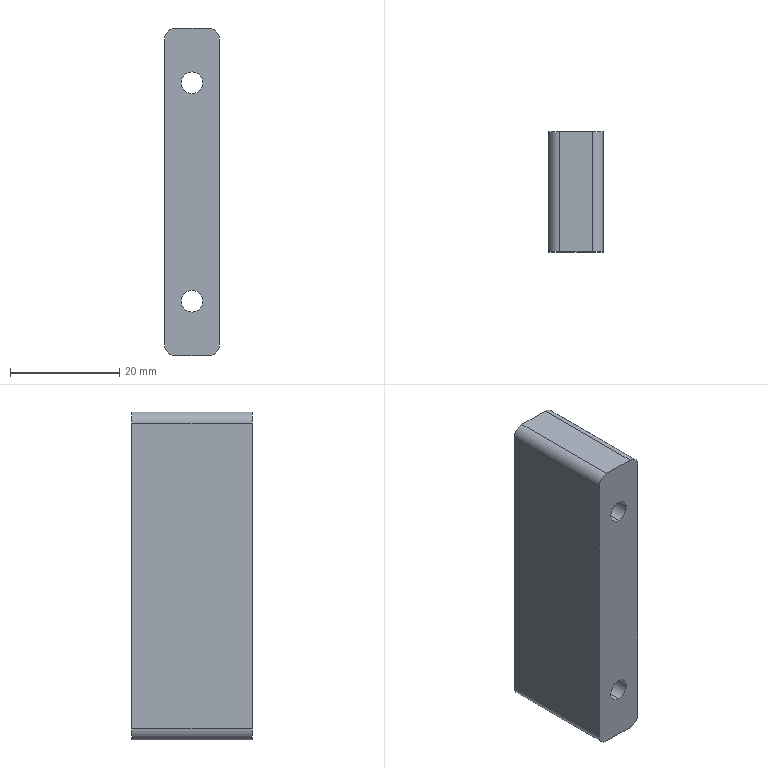Component | SolidWorks | Support-3 | 1 solid | 14 faces | box 10 x 22 x 60 mm | volume 12572 mm3 | cylinder 8 | plane 6 | commonest cylinder face diameters 4 x8
build123d program:
from build123d import *

# Parameters (mm, degrees)
SKETCH2_W           = 60
SKETCH2_H           = 10
SKETCH2_R           = 2
BOSS_EXTRUDE1_DEPTH = 22
FILLET1_R           = 2


with BuildPart() as part:
    # Sketch2 → Boss-Extrude1 (new body)
    with BuildSketch(Plane.XY):
        Rectangle(SKETCH2_W, SKETCH2_H)
        with Locations((-20, 0)):
            Circle(SKETCH2_R, mode=Mode.SUBTRACT)
        with Locations((20, 0)):
            Circle(SKETCH2_R, mode=Mode.SUBTRACT)
    extrude(amount=BOSS_EXTRUDE1_DEPTH)

    # Fillet1
    fillet1_edges = [part.edges().sort_by_distance(p)[0] for p in [
        (30, -5, 11),
        (-30, -5, 11),
        (-30, 5, 11),
        (30, 5, 11),
    ]]
    fillet(fillet1_edges, radius=FILLET1_R)


solid = part.part

# Placed as in the assembly
solid = solid.moved(Location((-141.534, 108.266, -166.507), (90, 0, 90)))
STEP:
#1=COLOUR_RGB('',0.7922,0.8196,0.9333);
#2=FILL_AREA_STYLE_COLOUR('',#1);
#3=FILL_AREA_STYLE('',(#2));
#4=SURFACE_STYLE_FILL_AREA(#3);
#5=SURFACE_SIDE_STYLE('',(#4));
#6=SURFACE_STYLE_USAGE(.BOTH.,#5);
#7=PRESENTATION_STYLE_ASSIGNMENT((#6));
#8=CARTESIAN_POINT('',(-5.572,4.262,-5.847));
#9=VERTEX_POINT('',#8);
#10=CARTESIAN_POINT('',(-5.572,4.262,-5.689));
#11=VERTEX_POINT('',#10);
#12=CARTESIAN_POINT('',(-5.572,4.262,-5.768));
#13=DIRECTION('',(0.,1.,0.));
#14=DIRECTION('',(0.,0.,1.));
#15=AXIS2_PLACEMENT_3D('',#12,#13,#14);
#16=CIRCLE('',#15,0.07874);
#17=EDGE_CURVE('',#9,#11,#16,.T.);
#18=ORIENTED_EDGE('',*,*,#17,.T.);
#19=CARTESIAN_POINT('',(-5.572,3.396,-5.689));
#20=VERTEX_POINT('',#19);
#21=CARTESIAN_POINT('',(-5.572,4.262,-5.689));
#22=DIRECTION('',(0.,-1.,0.));
#23=VECTOR('',#22,39.37);
#24=LINE('',#21,#23);
#25=EDGE_CURVE('',#11,#20,#24,.T.);
#26=ORIENTED_EDGE('',*,*,#25,.T.);
#27=CARTESIAN_POINT('',(-5.572,3.396,-5.847));
#28=VERTEX_POINT('',#27);
#29=CARTESIAN_POINT('',(-5.572,3.396,-5.768));
#30=DIRECTION('',(0.,1.,0.));
#31=DIRECTION('',(0.,0.,1.));
#32=AXIS2_PLACEMENT_3D('',#29,#30,#31);
#33=CIRCLE('',#32,0.07874);
#34=EDGE_CURVE('',#28,#20,#33,.T.);
#35=ORIENTED_EDGE('',*,*,#34,.F.);
#36=CARTESIAN_POINT('',(-5.572,4.262,-5.847));
#37=DIRECTION('',(0.,-1.,0.));
#38=VECTOR('',#37,39.37);
#39=LINE('',#36,#38);
#40=EDGE_CURVE('',#9,#28,#39,.T.);
#41=ORIENTED_EDGE('',*,*,#40,.F.);
#42=EDGE_LOOP('',(#18,#26,#35,#41));
#43=FACE_OUTER_BOUND('',#42,.T.);
#44=CARTESIAN_POINT('',(-5.572,4.262,-5.768));
#45=DIRECTION('',(0.,-1.,0.));
#46=DIRECTION('',(0.,0.,-1.));
#47=AXIS2_PLACEMENT_3D('',#44,#45,#46);
#48=CYLINDRICAL_SURFACE('',#47,0.07874);
#49=ADVANCED_FACE('',(#43),#48,.F.);
#50=CARTESIAN_POINT('',(-5.572,4.262,-7.422));
#51=VERTEX_POINT('',#50);
#52=CARTESIAN_POINT('',(-5.572,4.262,-7.264));
#53=VERTEX_POINT('',#52);
#54=CARTESIAN_POINT('',(-5.572,4.262,-7.343));
#55=DIRECTION('',(0.,1.,0.));
#56=DIRECTION('',(0.,0.,1.));
#57=AXIS2_PLACEMENT_3D('',#54,#55,#56);
#58=CIRCLE('',#57,0.07874);
#59=EDGE_CURVE('',#51,#53,#58,.T.);
#60=ORIENTED_EDGE('',*,*,#59,.T.);
#61=CARTESIAN_POINT('',(-5.572,3.396,-7.264));
#62=VERTEX_POINT('',#61);
#63=CARTESIAN_POINT('',(-5.572,4.262,-7.264));
#64=DIRECTION('',(0.,-1.,0.));
#65=VECTOR('',#64,39.37);
#66=LINE('',#63,#65);
#67=EDGE_CURVE('',#53,#62,#66,.T.);
#68=ORIENTED_EDGE('',*,*,#67,.T.);
#69=CARTESIAN_POINT('',(-5.572,3.396,-7.422));
#70=VERTEX_POINT('',#69);
#71=CARTESIAN_POINT('',(-5.572,3.396,-7.343));
#72=DIRECTION('',(0.,1.,0.));
#73=DIRECTION('',(0.,0.,1.));
#74=AXIS2_PLACEMENT_3D('',#71,#72,#73);
#75=CIRCLE('',#74,0.07874);
#76=EDGE_CURVE('',#70,#62,#75,.T.);
#77=ORIENTED_EDGE('',*,*,#76,.F.);
#78=CARTESIAN_POINT('',(-5.572,4.262,-7.422));
#79=DIRECTION('',(0.,-1.,0.));
#80=VECTOR('',#79,39.37);
#81=LINE('',#78,#80);
#82=EDGE_CURVE('',#51,#70,#81,.T.);
#83=ORIENTED_EDGE('',*,*,#82,.F.);
#84=EDGE_LOOP('',(#60,#68,#77,#83));
#85=FACE_OUTER_BOUND('',#84,.T.);
#86=CARTESIAN_POINT('',(-5.572,4.262,-7.343));
#87=DIRECTION('',(0.,-1.,0.));
#88=DIRECTION('',(0.,0.,-1.));
#89=AXIS2_PLACEMENT_3D('',#86,#87,#88);
#90=CYLINDRICAL_SURFACE('',#89,0.07874);
#91=ADVANCED_FACE('',(#85),#90,.F.);
#92=ORIENTED_EDGE('',*,*,#59,.F.);
#93=CARTESIAN_POINT('',(-5.572,4.262,-7.343));
#94=DIRECTION('',(0.,1.,0.));
#95=DIRECTION('',(0.,0.,1.));
#96=AXIS2_PLACEMENT_3D('',#93,#94,#95);
#97=CIRCLE('',#96,0.07874);
#98=EDGE_CURVE('',#53,#51,#97,.T.);
#99=ORIENTED_EDGE('',*,*,#98,.F.);
#100=EDGE_LOOP('',(#92,#99));
#101=FACE_BOUND('',#100,.T.);
#102=CARTESIAN_POINT('',(-5.375,4.262,-5.453));
#103=VERTEX_POINT('',#102);
#104=CARTESIAN_POINT('',(-5.375,4.262,-7.658));
#105=VERTEX_POINT('',#104);
#106=CARTESIAN_POINT('',(-5.375,4.262,-7.736));
#107=DIRECTION('',(0.,0.,-1.));
#108=VECTOR('',#107,39.37);
#109=LINE('',#106,#108);
#110=EDGE_CURVE('',#103,#105,#109,.T.);
#111=ORIENTED_EDGE('',*,*,#110,.T.);
#112=CARTESIAN_POINT('',(-5.454,4.262,-7.736));
#113=VERTEX_POINT('',#112);
#114=CARTESIAN_POINT('',(-5.454,4.262,-7.658));
#115=DIRECTION('',(0.,1.,0.));
#116=DIRECTION('',(0.,0.,1.));
#117=AXIS2_PLACEMENT_3D('',#114,#115,#116);
#118=CIRCLE('',#117,0.07874);
#119=EDGE_CURVE('',#105,#113,#118,.T.);
#120=ORIENTED_EDGE('',*,*,#119,.T.);
#121=CARTESIAN_POINT('',(-5.69,4.262,-7.736));
#122=VERTEX_POINT('',#121);
#123=CARTESIAN_POINT('',(-5.375,4.262,-7.736));
#124=DIRECTION('',(-1.,0.,-0.));
#125=VECTOR('',#124,39.37);
#126=LINE('',#123,#125);
#127=EDGE_CURVE('',#113,#122,#126,.T.);
#128=ORIENTED_EDGE('',*,*,#127,.T.);
#129=CARTESIAN_POINT('',(-5.769,4.262,-7.658));
#130=VERTEX_POINT('',#129);
#131=CARTESIAN_POINT('',(-5.69,4.262,-7.658));
#132=DIRECTION('',(0.,1.,0.));
#133=DIRECTION('',(0.,0.,1.));
#134=AXIS2_PLACEMENT_3D('',#131,#132,#133);
#135=CIRCLE('',#134,0.07874);
#136=EDGE_CURVE('',#122,#130,#135,.T.);
#137=ORIENTED_EDGE('',*,*,#136,.T.);
#138=CARTESIAN_POINT('',(-5.769,4.262,-5.453));
#139=VERTEX_POINT('',#138);
#140=CARTESIAN_POINT('',(-5.769,4.262,-7.736));
#141=DIRECTION('',(-0.,0.,1.));
#142=VECTOR('',#141,39.37);
#143=LINE('',#140,#142);
#144=EDGE_CURVE('',#130,#139,#143,.T.);
#145=ORIENTED_EDGE('',*,*,#144,.T.);
#146=CARTESIAN_POINT('',(-5.69,4.262,-5.374));
#147=VERTEX_POINT('',#146);
#148=CARTESIAN_POINT('',(-5.69,4.262,-5.453));
#149=DIRECTION('',(0.,1.,0.));
#150=DIRECTION('',(0.,0.,1.));
#151=AXIS2_PLACEMENT_3D('',#148,#149,#150);
#152=CIRCLE('',#151,0.07874);
#153=EDGE_CURVE('',#139,#147,#152,.T.);
#154=ORIENTED_EDGE('',*,*,#153,.T.);
#155=CARTESIAN_POINT('',(-5.454,4.262,-5.374));
#156=VERTEX_POINT('',#155);
#157=CARTESIAN_POINT('',(-5.375,4.262,-5.374));
#158=DIRECTION('',(1.,0.,0.));
#159=VECTOR('',#158,39.37);
#160=LINE('',#157,#159);
#161=EDGE_CURVE('',#147,#156,#160,.T.);
#162=ORIENTED_EDGE('',*,*,#161,.T.);
#163=CARTESIAN_POINT('',(-5.454,4.262,-5.453));
#164=DIRECTION('',(0.,1.,0.));
#165=DIRECTION('',(0.,0.,1.));
#166=AXIS2_PLACEMENT_3D('',#163,#164,#165);
#167=CIRCLE('',#166,0.07874);
#168=EDGE_CURVE('',#156,#103,#167,.T.);
#169=ORIENTED_EDGE('',*,*,#168,.T.);
#170=EDGE_LOOP('',(#111,#120,#128,#137,#145,#154,#162,#169));
#171=FACE_OUTER_BOUND('',#170,.T.);
#172=ORIENTED_EDGE('',*,*,#17,.F.);
#173=CARTESIAN_POINT('',(-5.572,4.262,-5.768));
#174=DIRECTION('',(0.,1.,0.));
#175=DIRECTION('',(0.,0.,1.));
#176=AXIS2_PLACEMENT_3D('',#173,#174,#175);
#177=CIRCLE('',#176,0.07874);
#178=EDGE_CURVE('',#11,#9,#177,.T.);
#179=ORIENTED_EDGE('',*,*,#178,.F.);
#180=EDGE_LOOP('',(#172,#179));
#181=FACE_BOUND('',#180,.T.);
#182=CARTESIAN_POINT('',(-5.572,4.262,-6.555));
#183=DIRECTION('',(0.,1.,0.));
#184=DIRECTION('',(-0.,0.,1.));
#185=AXIS2_PLACEMENT_3D('',#182,#183,#184);
#186=PLANE('',#185);
#187=ADVANCED_FACE('',(#101,#171,#181),#186,.T.);
#188=CARTESIAN_POINT('',(-5.454,3.396,-7.736));
#189=VERTEX_POINT('',#188);
#190=CARTESIAN_POINT('',(-5.69,3.396,-7.736));
#191=VERTEX_POINT('',#190);
#192=CARTESIAN_POINT('',(-5.375,3.396,-7.736));
#193=DIRECTION('',(-1.,0.,-0.));
#194=VECTOR('',#193,39.37);
#195=LINE('',#192,#194);
#196=EDGE_CURVE('',#189,#191,#195,.T.);
#197=ORIENTED_EDGE('',*,*,#196,.F.);
#198=CARTESIAN_POINT('',(-5.375,3.396,-7.658));
#199=VERTEX_POINT('',#198);
#200=CARTESIAN_POINT('',(-5.454,3.396,-7.658));
#201=DIRECTION('',(0.,-1.,0.));
#202=DIRECTION('',(0.,0.,1.));
#203=AXIS2_PLACEMENT_3D('',#200,#201,#202);
#204=CIRCLE('',#203,0.07874);
#205=EDGE_CURVE('',#189,#199,#204,.T.);
#206=ORIENTED_EDGE('',*,*,#205,.T.);
#207=CARTESIAN_POINT('',(-5.375,3.396,-5.453));
#208=VERTEX_POINT('',#207);
#209=CARTESIAN_POINT('',(-5.375,3.396,-7.736));
#210=DIRECTION('',(0.,0.,-1.));
#211=VECTOR('',#210,39.37);
#212=LINE('',#209,#211);
#213=EDGE_CURVE('',#208,#199,#212,.T.);
#214=ORIENTED_EDGE('',*,*,#213,.F.);
#215=CARTESIAN_POINT('',(-5.454,3.396,-5.374));
#216=VERTEX_POINT('',#215);
#217=CARTESIAN_POINT('',(-5.454,3.396,-5.453));
#218=DIRECTION('',(0.,-1.,0.));
#219=DIRECTION('',(0.,0.,1.));
#220=AXIS2_PLACEMENT_3D('',#217,#218,#219);
#221=CIRCLE('',#220,0.07874);
#222=EDGE_CURVE('',#208,#216,#221,.T.);
#223=ORIENTED_EDGE('',*,*,#222,.T.);
#224=CARTESIAN_POINT('',(-5.69,3.396,-5.374));
#225=VERTEX_POINT('',#224);
#226=CARTESIAN_POINT('',(-5.375,3.396,-5.374));
#227=DIRECTION('',(1.,0.,0.));
#228=VECTOR('',#227,39.37);
#229=LINE('',#226,#228);
#230=EDGE_CURVE('',#225,#216,#229,.T.);
#231=ORIENTED_EDGE('',*,*,#230,.F.);
#232=CARTESIAN_POINT('',(-5.769,3.396,-5.453));
#233=VERTEX_POINT('',#232);
#234=CARTESIAN_POINT('',(-5.69,3.396,-5.453));
#235=DIRECTION('',(0.,-1.,0.));
#236=DIRECTION('',(0.,0.,1.));
#237=AXIS2_PLACEMENT_3D('',#234,#235,#236);
#238=CIRCLE('',#237,0.07874);
#239=EDGE_CURVE('',#225,#233,#238,.T.);
#240=ORIENTED_EDGE('',*,*,#239,.T.);
#241=CARTESIAN_POINT('',(-5.769,3.396,-7.658));
#242=VERTEX_POINT('',#241);
#243=CARTESIAN_POINT('',(-5.769,3.396,-7.736));
#244=DIRECTION('',(-0.,0.,1.));
#245=VECTOR('',#244,39.37);
#246=LINE('',#243,#245);
#247=EDGE_CURVE('',#242,#233,#246,.T.);
#248=ORIENTED_EDGE('',*,*,#247,.F.);
#249=CARTESIAN_POINT('',(-5.69,3.396,-7.658));
#250=DIRECTION('',(0.,-1.,0.));
#251=DIRECTION('',(0.,0.,1.));
#252=AXIS2_PLACEMENT_3D('',#249,#250,#251);
#253=CIRCLE('',#252,0.07874);
#254=EDGE_CURVE('',#242,#191,#253,.T.);
#255=ORIENTED_EDGE('',*,*,#254,.T.);
#256=EDGE_LOOP('',(#197,#206,#214,#223,#231,#240,#248,#255));
#257=FACE_OUTER_BOUND('',#256,.T.);
#258=ORIENTED_EDGE('',*,*,#76,.T.);
#259=CARTESIAN_POINT('',(-5.572,3.396,-7.343));
#260=DIRECTION('',(0.,1.,0.));
#261=DIRECTION('',(0.,0.,1.));
#262=AXIS2_PLACEMENT_3D('',#259,#260,#261);
#263=CIRCLE('',#262,0.07874);
#264=EDGE_CURVE('',#62,#70,#263,.T.);
#265=ORIENTED_EDGE('',*,*,#264,.T.);
#266=EDGE_LOOP('',(#258,#265));
#267=FACE_BOUND('',#266,.T.);
#268=ORIENTED_EDGE('',*,*,#34,.T.);
#269=CARTESIAN_POINT('',(-5.572,3.396,-5.768));
#270=DIRECTION('',(0.,1.,0.));
#271=DIRECTION('',(0.,0.,1.));
#272=AXIS2_PLACEMENT_3D('',#269,#270,#271);
#273=CIRCLE('',#272,0.07874);
#274=EDGE_CURVE('',#20,#28,#273,.T.);
#275=ORIENTED_EDGE('',*,*,#274,.T.);
#276=EDGE_LOOP('',(#268,#275));
#277=FACE_BOUND('',#276,.T.);
#278=CARTESIAN_POINT('',(-5.572,3.396,-6.555));
#279=DIRECTION('',(0.,1.,0.));
#280=DIRECTION('',(-0.,0.,1.));
#281=AXIS2_PLACEMENT_3D('',#278,#279,#280);
#282=PLANE('',#281);
#283=ADVANCED_FACE('',(#257,#267,#277),#282,.F.);
#284=ORIENTED_EDGE('',*,*,#161,.F.);
#285=CARTESIAN_POINT('',(-5.69,4.262,-5.374));
#286=DIRECTION('',(0.,-1.,0.));
#287=VECTOR('',#286,39.37);
#288=LINE('',#285,#287);
#289=EDGE_CURVE('',#147,#225,#288,.T.);
#290=ORIENTED_EDGE('',*,*,#289,.T.);
#291=ORIENTED_EDGE('',*,*,#230,.T.);
#292=CARTESIAN_POINT('',(-5.454,4.262,-5.374));
#293=DIRECTION('',(0.,1.,0.));
#294=VECTOR('',#293,39.37);
#295=LINE('',#292,#294);
#296=EDGE_CURVE('',#216,#156,#295,.T.);
#297=ORIENTED_EDGE('',*,*,#296,.T.);
#298=EDGE_LOOP('',(#284,#290,#291,#297));
#299=FACE_OUTER_BOUND('',#298,.T.);
#300=CARTESIAN_POINT('',(-5.375,4.262,-5.374));
#301=DIRECTION('',(0.,0.,-1.));
#302=DIRECTION('',(0.,1.,0.));
#303=AXIS2_PLACEMENT_3D('',#300,#301,#302);
#304=PLANE('',#303);
#305=ADVANCED_FACE('',(#299),#304,.F.);
#306=ORIENTED_EDGE('',*,*,#213,.T.);
#307=CARTESIAN_POINT('',(-5.375,4.262,-7.658));
#308=DIRECTION('',(0.,1.,0.));
#309=VECTOR('',#308,39.37);
#310=LINE('',#307,#309);
#311=EDGE_CURVE('',#199,#105,#310,.T.);
#312=ORIENTED_EDGE('',*,*,#311,.T.);
#313=ORIENTED_EDGE('',*,*,#110,.F.);
#314=CARTESIAN_POINT('',(-5.375,4.262,-5.453));
#315=DIRECTION('',(0.,-1.,0.));
#316=VECTOR('',#315,39.37);
#317=LINE('',#314,#316);
#318=EDGE_CURVE('',#103,#208,#317,.T.);
#319=ORIENTED_EDGE('',*,*,#318,.T.);
#320=EDGE_LOOP('',(#306,#312,#313,#319));
#321=FACE_OUTER_BOUND('',#320,.T.);
#322=CARTESIAN_POINT('',(-5.375,4.262,-7.736));
#323=DIRECTION('',(-1.,0.,-0.));
#324=DIRECTION('',(0.,-1.,0.));
#325=AXIS2_PLACEMENT_3D('',#322,#323,#324);
#326=PLANE('',#325);
#327=ADVANCED_FACE('',(#321),#326,.F.);
#328=ORIENTED_EDGE('',*,*,#127,.F.);
#329=CARTESIAN_POINT('',(-5.454,4.262,-7.736));
#330=DIRECTION('',(0.,-1.,0.));
#331=VECTOR('',#330,39.37);
#332=LINE('',#329,#331);
#333=EDGE_CURVE('',#113,#189,#332,.T.);
#334=ORIENTED_EDGE('',*,*,#333,.T.);
#335=ORIENTED_EDGE('',*,*,#196,.T.);
#336=CARTESIAN_POINT('',(-5.69,4.262,-7.736));
#337=DIRECTION('',(0.,1.,0.));
#338=VECTOR('',#337,39.37);
#339=LINE('',#336,#338);
#340=EDGE_CURVE('',#191,#122,#339,.T.);
#341=ORIENTED_EDGE('',*,*,#340,.T.);
#342=EDGE_LOOP('',(#328,#334,#335,#341));
#343=FACE_OUTER_BOUND('',#342,.T.);
#344=CARTESIAN_POINT('',(-5.375,4.262,-7.736));
#345=DIRECTION('',(-0.,0.,1.));
#346=DIRECTION('',(0.,-1.,0.));
#347=AXIS2_PLACEMENT_3D('',#344,#345,#346);
#348=PLANE('',#347);
#349=ADVANCED_FACE('',(#343),#348,.F.);
#350=ORIENTED_EDGE('',*,*,#247,.T.);
#351=CARTESIAN_POINT('',(-5.769,4.262,-5.453));
#352=DIRECTION('',(0.,1.,0.));
#353=VECTOR('',#352,39.37);
#354=LINE('',#351,#353);
#355=EDGE_CURVE('',#233,#139,#354,.T.);
#356=ORIENTED_EDGE('',*,*,#355,.T.);
#357=ORIENTED_EDGE('',*,*,#144,.F.);
#358=CARTESIAN_POINT('',(-5.769,4.262,-7.658));
#359=DIRECTION('',(0.,-1.,0.));
#360=VECTOR('',#359,39.37);
#361=LINE('',#358,#360);
#362=EDGE_CURVE('',#130,#242,#361,.T.);
#363=ORIENTED_EDGE('',*,*,#362,.T.);
#364=EDGE_LOOP('',(#350,#356,#357,#363));
#365=FACE_OUTER_BOUND('',#364,.T.);
#366=CARTESIAN_POINT('',(-5.769,4.262,-7.736));
#367=DIRECTION('',(1.,0.,0.));
#368=DIRECTION('',(0.,1.,0.));
#369=AXIS2_PLACEMENT_3D('',#366,#367,#368);
#370=PLANE('',#369);
#371=ADVANCED_FACE('',(#365),#370,.F.);
#372=ORIENTED_EDGE('',*,*,#67,.F.);
#373=ORIENTED_EDGE('',*,*,#98,.T.);
#374=ORIENTED_EDGE('',*,*,#82,.T.);
#375=ORIENTED_EDGE('',*,*,#264,.F.);
#376=EDGE_LOOP('',(#372,#373,#374,#375));
#377=FACE_OUTER_BOUND('',#376,.T.);
#378=CARTESIAN_POINT('',(-5.572,4.262,-7.343));
#379=DIRECTION('',(0.,-1.,0.));
#380=DIRECTION('',(0.,0.,-1.));
#381=AXIS2_PLACEMENT_3D('',#378,#379,#380);
#382=CYLINDRICAL_SURFACE('',#381,0.07874);
#383=ADVANCED_FACE('',(#377),#382,.F.);
#384=ORIENTED_EDGE('',*,*,#25,.F.);
#385=ORIENTED_EDGE('',*,*,#178,.T.);
#386=ORIENTED_EDGE('',*,*,#40,.T.);
#387=ORIENTED_EDGE('',*,*,#274,.F.);
#388=EDGE_LOOP('',(#384,#385,#386,#387));
#389=FACE_OUTER_BOUND('',#388,.T.);
#390=CARTESIAN_POINT('',(-5.572,4.262,-5.768));
#391=DIRECTION('',(0.,-1.,0.));
#392=DIRECTION('',(0.,0.,-1.));
#393=AXIS2_PLACEMENT_3D('',#390,#391,#392);
#394=CYLINDRICAL_SURFACE('',#393,0.07874);
#395=ADVANCED_FACE('',(#389),#394,.F.);
#396=ORIENTED_EDGE('',*,*,#119,.F.);
#397=ORIENTED_EDGE('',*,*,#311,.F.);
#398=ORIENTED_EDGE('',*,*,#205,.F.);
#399=ORIENTED_EDGE('',*,*,#333,.F.);
#400=EDGE_LOOP('',(#396,#397,#398,#399));
#401=FACE_OUTER_BOUND('',#400,.T.);
#402=CARTESIAN_POINT('',(-5.454,4.262,-7.658));
#403=DIRECTION('',(0.,-1.,0.));
#404=DIRECTION('',(0.,0.,-1.));
#405=AXIS2_PLACEMENT_3D('',#402,#403,#404);
#406=CYLINDRICAL_SURFACE('',#405,0.07874);
#407=ADVANCED_FACE('',(#401),#406,.T.);
#408=ORIENTED_EDGE('',*,*,#153,.F.);
#409=ORIENTED_EDGE('',*,*,#355,.F.);
#410=ORIENTED_EDGE('',*,*,#239,.F.);
#411=ORIENTED_EDGE('',*,*,#289,.F.);
#412=EDGE_LOOP('',(#408,#409,#410,#411));
#413=FACE_OUTER_BOUND('',#412,.T.);
#414=CARTESIAN_POINT('',(-5.69,4.262,-5.453));
#415=DIRECTION('',(0.,-1.,0.));
#416=DIRECTION('',(0.,0.,-1.));
#417=AXIS2_PLACEMENT_3D('',#414,#415,#416);
#418=CYLINDRICAL_SURFACE('',#417,0.07874);
#419=ADVANCED_FACE('',(#413),#418,.T.);
#420=ORIENTED_EDGE('',*,*,#136,.F.);
#421=ORIENTED_EDGE('',*,*,#340,.F.);
#422=ORIENTED_EDGE('',*,*,#254,.F.);
#423=ORIENTED_EDGE('',*,*,#362,.F.);
#424=EDGE_LOOP('',(#420,#421,#422,#423));
#425=FACE_OUTER_BOUND('',#424,.T.);
#426=CARTESIAN_POINT('',(-5.69,4.262,-7.658));
#427=DIRECTION('',(0.,-1.,0.));
#428=DIRECTION('',(0.,0.,-1.));
#429=AXIS2_PLACEMENT_3D('',#426,#427,#428);
#430=CYLINDRICAL_SURFACE('',#429,0.07874);
#431=ADVANCED_FACE('',(#425),#430,.T.);
#432=ORIENTED_EDGE('',*,*,#168,.F.);
#433=ORIENTED_EDGE('',*,*,#296,.F.);
#434=ORIENTED_EDGE('',*,*,#222,.F.);
#435=ORIENTED_EDGE('',*,*,#318,.F.);
#436=EDGE_LOOP('',(#432,#433,#434,#435));
#437=FACE_OUTER_BOUND('',#436,.T.);
#438=CARTESIAN_POINT('',(-5.454,4.262,-5.453));
#439=DIRECTION('',(0.,-1.,0.));
#440=DIRECTION('',(0.,0.,-1.));
#441=AXIS2_PLACEMENT_3D('',#438,#439,#440);
#442=CYLINDRICAL_SURFACE('',#441,0.07874);
#443=ADVANCED_FACE('',(#437),#442,.T.);
#444=CLOSED_SHELL('',(#49,#91,#187,#283,#305,#327,#349,#371,#383,#395,#407,#419,#431,#443));
#445=MANIFOLD_SOLID_BREP('',#444);
#446=STYLED_ITEM('',(#7),#445);
#447=PRESENTATION_LAYER_ASSIGNMENT('','',(#446));
#448=CARTESIAN_POINT('',(0.,0.,0.));
#449=DIRECTION('',(0.,0.,1.));
#450=DIRECTION('',(1.,0.,0.));
#451=AXIS2_PLACEMENT_3D('',#448,#449,#450);
#452=(LENGTH_UNIT()NAMED_UNIT(*)SI_UNIT($,.METRE.));
#453=LENGTH_MEASURE_WITH_UNIT(LENGTH_MEASURE(0.0254),#452);
#454=DIMENSIONAL_EXPONENTS(1.,0.,0.,0.,0.,0.,0.);
#455=(CONVERSION_BASED_UNIT('',#453)LENGTH_UNIT()NAMED_UNIT(#454));
#456=UNCERTAINTY_MEASURE_WITH_UNIT(LENGTH_MEASURE(0.00001),#455,'','');
#457=(NAMED_UNIT(*)PLANE_ANGLE_UNIT()SI_UNIT($,.RADIAN.));
#458=(NAMED_UNIT(*)SI_UNIT($,.STERADIAN.)SOLID_ANGLE_UNIT());
#459=(GEOMETRIC_REPRESENTATION_CONTEXT(3)GLOBAL_UNCERTAINTY_ASSIGNED_CONTEXT((#456))GLOBAL_UNIT_ASSIGNED_CONTEXT((#455,#457,#458))REPRESENTATION_CONTEXT('',''));
#460=ADVANCED_BREP_SHAPE_REPRESENTATION('',(#445,#451),#459);
#461=(LENGTH_UNIT()NAMED_UNIT(*)SI_UNIT($,.METRE.));
#462=LENGTH_MEASURE_WITH_UNIT(LENGTH_MEASURE(0.0254),#461);
#463=DIMENSIONAL_EXPONENTS(1.,0.,0.,0.,0.,0.,0.);
#464=(CONVERSION_BASED_UNIT('',#462)LENGTH_UNIT()NAMED_UNIT(#463));
#465=UNCERTAINTY_MEASURE_WITH_UNIT(LENGTH_MEASURE(0.00001),#464,'','');
#466=(NAMED_UNIT(*)PLANE_ANGLE_UNIT()SI_UNIT($,.RADIAN.));
#467=(NAMED_UNIT(*)SI_UNIT($,.STERADIAN.)SOLID_ANGLE_UNIT());
#468=(GEOMETRIC_REPRESENTATION_CONTEXT(3)GLOBAL_UNCERTAINTY_ASSIGNED_CONTEXT((#465))GLOBAL_UNIT_ASSIGNED_CONTEXT((#464,#466,#467))REPRESENTATION_CONTEXT('',''));
#469=MECHANICAL_DESIGN_GEOMETRIC_PRESENTATION_REPRESENTATION('',(#446),#468);